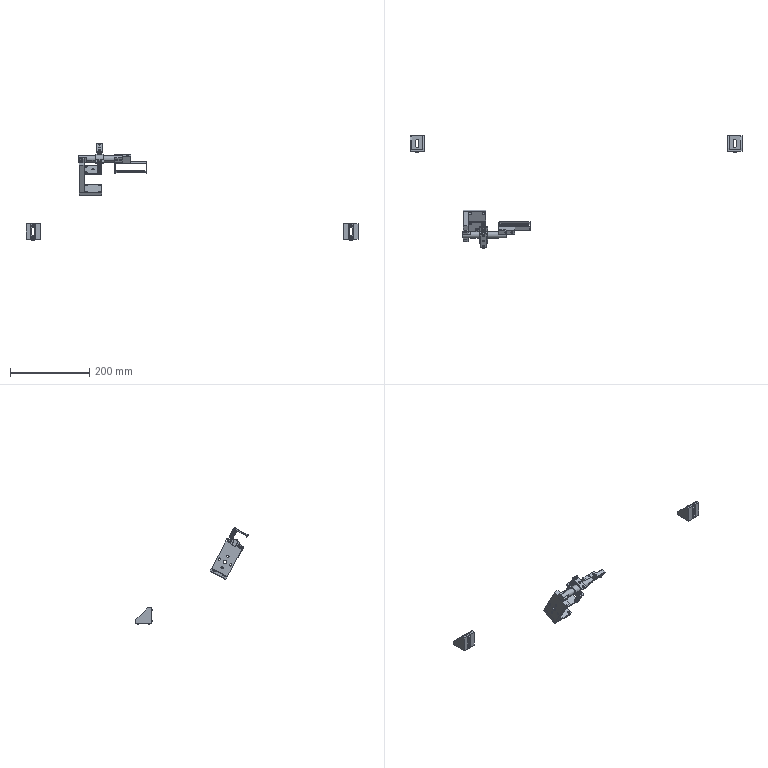Assembly | SolidWorks | mm | 21 component files | 21 solids | 520 faces | box 836 x 284.58 x 242.95 mm | volume 129529 mm3 | plane 300 | cylinder 172 | cone 24 | torus 18 | spline 6 | commonest cylinder face diameters 6 x22 10 x14 5 x12 4 x12 5.5 x12 6.5 x12 3 x10 7 x10
Bill of materials:
ABB11-G408-4040AngleBracket | 2 |  | Right-angle corner-block bracket with a triangular, chamfered side profile. Each of its two perpendicular faces has an obround slot, and small rectangular locating tabs stick out from those faces.
BladeConnectingRod | 1 |  | Solid cylindrical shaft or rod with a flat milled on each end. One flat has a single larger cross hole; the other has two smaller holes.
clevis pins with head gb | 1 |  | Headed cylindrical pin with a domed, rounded head, a plain shank, and one transverse cross hole near the chamfered tip, consistent with a clevis-style pin.
hexagon socket head cap screws gb | 4 |  | Socket-head cap-screw-shaped part: a cylindrical head with a hexagonal socket and a plain cylindrical shank.
RotaryCylinderFixingPlate | 1 |  | Thick rectangular plate or block with two narrow tabs extending from one edge, each with a hole through its thickness. The main face has a pattern of one larger centre hole and four smaller surrounding holes.
SDACylinderFixingPlate | 1 |  | Flat rectangular plate with sharp corners and six through-holes in two rows of three. The holes near one edge are smaller than the others.
SDACylinderPushPlate | 1 |  | Thin flat rectangular plate with rounded corners, four corner through-holes and one larger central through-hole.
SDACylinderSpringPressurePlate | 1 |  | Flat elongated strip/link plate with rounded corners: two larger through-holes near the ends and one smaller through-hole at the centre.
split pins | 1 |  | Split pin (cotter-pin-like) shape: a wire folded back on itself, with a looped eye at one end and two legs of unequal length with flat inner faces.
Spring | 2 |  | Helical coil spring with round wire, constant diameter and open, evenly spaced coils.
Spring | 1 |  | Open-coiled cylindrical helix shaped like a coil spring: a single continuous wire wound at a constant coil diameter and roughly even pitch, about 11-12 turns, with plain cut ends.
SpringSnap | 2 |  | Formed sheet-metal saddle/pipe-clamp shape: a central semicircular arch with flat flanges on both sides, each flange having an obround slot.
Blade | 1 |  | Long, narrow bent sheet strip with a V-shaped end profile and a rounded bend. A long rectangular opening runs along most of its length, and small narrow tabs extend at each end.
CutterFixingBlock | 1 |  | Solid rectangular block with sharp edges. It has two round holes in one long face and two round holes in an adjacent perpendicular face. One hole from each pair breaks into a hole from the other pair.
ToolHolder | 1 |  | Strap of thin bent sheet with a U or channel shape. A long flat middle section has two round holes and is bent at both ends into legs on the same side. Each leg narrows to a rounded tip with one small round hole.
Mates:
1. coincident | RotaryCylinderFixingPlate-1 face at (-267.317, -3.29, 87.691) dir (0, 0.4648, -0.8854) | SDACylinderFixingPlate-1 face at (-251.317, 16.632, 98.15) dir (0, -0.4648, 0.8854)
2. coincident | RotaryCylinderFixingPlate-1 face at (-267.317, -5.28, 188.295) dir (0, 0.8854, 0.4648) | SDACylinderFixingPlate-1 face at (-223.317, 40.272, 101.525) dir (0, 0.8854, 0.4648)
3. coincident | RotaryCylinderFixingPlate-1 face at (-279.317, -4.285, 137.993) dir (-1, 0, 0) | SDACylinderFixingPlate-1 face at (-279.317, 0.429, 80.608) dir (-1, 0, 0)
4. coincident | RotaryCylinderFixingPlate-1 face at (-279.317, -36.136, 187.908) dir (0, 0.8854, 0.4648) | BladeConnectingRod-1 face at (-260.317, -23.937, 164.67) dir (0, -0.8854, -0.4648)
5. concentric | RotaryCylinderFixingPlate-1 face at (-273.317, -13.559, 177.172) dir (0, 0.8854, 0.4648) r 3 | BladeConnectingRod-1 face at (-273.317, -26.84, 170.2) dir (0, -0.8854, -0.4648) r 3
6. concentric | ToolHolderAssembly-1/CutterFixingBlock-1 face at (-185.317, -17.986, 174.848) dir (0, -0.8854, -0.4648) r 2.5 | BladeConnectingRod-1 face at (-185.317, -26.84, 170.2) dir (0, -0.8854, -0.4648) r 1.65
7. concentric | ToolHolderAssembly-1/CutterFixingBlock-1 face at (-175.317, -17.986, 174.848) dir (0, -0.8854, -0.4648) r 2.5 | BladeConnectingRod-1 face at (-175.317, -26.84, 170.2) dir (0, -0.8854, -0.4648) r 1.65
8. parallel | RotaryCylinderFixingPlate-1 face at (-267.317, -5.28, 188.295) dir (0, 0.8854, 0.4648) | SDACylinderPushPlate-1 face at (-223.317, 9.286, 155.17) dir (0, 0.8854, 0.4648)
9. concentric | SDACylinderPushPlate-1 face at (-228.317, -20.308, 136.245) dir (0, 0.4648, -0.8854) r 2.5 | SDACylinderSpringPressurePlate-1 face at (-228.317, -50.986, 194.681) dir (0, -0.4648, 0.8854) r 3.25
10. distance | SDACylinderPushPlate-1 face at (-245.317, -8.422, 145.873) dir (0, -0.4648, 0.8854) | SDACylinderSpringPressurePlate-1 face at (-228.317, -36.311, 198.998) dir (0, 0.4648, -0.8854)
11. concentric | hexagon socket head cap screws gb-2 face at (-228.317, -21.635, 203.314) dir (0, -0.4648, 0.8854) r 0.8 | SDACylinderSpringPressurePlate-1 face at (-228.317, -24.424, 208.626) dir (0, -0.4648, 0.8854) r 3.25
12. coincident | SDACylinderSpringPressurePlate-1 face at (-228.317, -37.705, 201.654) dir (0, -0.4648, 0.8854) | hexagon socket head cap screws gb-2 face at (-228.317, -24.424, 208.626) dir (0, 0.4648, -0.8854)
13. concentric | SDACylinderPushPlate-1 face at (-228.317, 6.254, 150.189) dir (0, 0.4648, -0.8854) r 2.5 | hexagon socket head cap screws gb-2 face at (-228.317, -21.635, 203.314) dir (0, -0.4648, 0.8854) r 0.8
14. slot | SpringSnap-1 face at (-225.822, -2.314, 174.04) dir (0, -0.8854, -0.4648) | hexagon socket head cap screws gb-2 face at (-228.317, -21.635, 203.314) dir (0, -0.4648, 0.8854) r 0.8
15. slot | SpringSnap-1 face at (-226.423, -35.074, 156.842) dir (0, 0.8854, 0.4648) | hexagon socket head cap screws gb-3 face at (-228.317, -51.739, 187.51) dir (0, -0.4648, 0.8854) r 0.8
16. coincident | SpringSnap-1 face at (-218.322, -29.496, 168.805) dir (0, 0.4648, -0.8854) | SpringSnap-2 face at (-238.322, -15.329, 176.242) dir (0, -0.4648, 0.8854)
17. coincident | SpringSnap-1 face at (-218.322, -42.777, 161.833) dir (0, -0.8854, -0.4648) | SpringSnap-2 face at (-238.322, -42.777, 161.833) dir (0, -0.8854, -0.4648)
18. coincident | SpringSnap-1 face at (-218.322, -32.159, 170.286) dir (1, 0, 0) | SpringSnap-2 face at (-218.322, -30.333, 165.275) dir (1, 0, 0)
19. coincident | ToolHolderAssembly-1/CutterFixingBlock-1 face at (-150.317, -20.45, 179.542) dir (0, -0.8854, -0.4648) | BladeConnectingRod-1 face at (-190.317, -15.083, 169.319) dir (0, 0.8854, 0.4648)
20. concentric | BladeConnectingRod-1 face at (-273.317, -26.84, 170.2) dir (0, -0.8854, -0.4648) r 3 | clevis pins with head gb-1 face at (-273.317, 5.327, 187.087) dir (0, 0.8854, 0.4648) r 1.5
21. coincident | RotaryCylinderFixingPlate-1 face at (-279.317, -16.348, 182.485) dir (0, 0.8854, 0.4648) | clevis pins with head gb-1 face at (-274.637, -13.889, 177.802) dir (0, -0.8854, -0.4648)
22. concentric | clevis pins with head gb-1 face at (-271.115, -20.091, 172.404) dir (-0.8805, -0.2203, 0.4197) r 0.87 | split pins-2 face at (-262.72, -17.99, 168.403) dir (-0.8805, -0.2203, 0.4197) r 0.25
23. concentric | hexagon socket head cap screws gb-2 face at (-228.317, -21.635, 203.314) dir (0, -0.4648, 0.8854) r 0.8 | Spring-1 sketch segment at (-228.317, 4.976, 152.623) dir (0, -0.4648, 0.8854) r 4.5
24. coincident | SDACylinderPushPlate-1 face at (-245.317, -8.422, 145.873) dir (0, -0.4648, 0.8854) | Spring-1 face at (-237.317, -0.1812, 150.199) dir (0, 0.4648, -0.8854)
25. concentric | hexagon socket head cap screws gb-3 face at (-228.317, -51.739, 187.51) dir (0, -0.4648, 0.8854) r 0.8 | Spring-2 sketch segment at (-228.317, -25.128, 136.819) dir (0, -0.4648, 0.8854) r 4.5
26. coincident | SDACylinderPushPlate-1 face at (-245.317, -8.422, 145.873) dir (0, -0.4648, 0.8854) | Spring-2 face at (-237.317, -30.285, 134.395) dir (0, 0.4648, -0.8854)
27. concentric | hexagon socket head cap screws gb-2 face at (-228.317, -21.635, 203.314) dir (0, -0.4648, 0.8854) r 0.8 | Spring-3 sketch segment at (-228.317, -23.146, 206.192) dir (0, 0.4648, -0.8854) r 4.5
28. coincident | SDACylinderSpringPressurePlate-1 face at (-228.317, -36.311, 198.998) dir (0, 0.4648, -0.8854) | Spring-3 face at (-238.89, -23.98, 205.471) dir (0, -0.4648, 0.8854)
29. concentric | BladeConnectingRod-1 face at (-170.317, -22.413, 172.524) dir (-1, 0, 0) r 8 | SpringSnap-1 face at (-218.322, -22.413, 172.524) dir (-1, 0, 0) r 8
30. tangent | RotaryCylinderFixingPlate-1 face at (-279.317, -23.121, 163.117) dir (0, -0.4648, 0.8854) | BladeConnectingRod-1 face at (-170.317, -22.413, 172.524) dir (-1, 0, 0) r 8
31. concentric | Blade-1 face at (-29.739, 17.848, 39.396) dir (0, 0, -1) r 1.25 | ToolHolder-1 face at (-29.739, 17.848, -41.604) dir (0, 0, 1) r 1.25
32. coincident | Blade-1 face at (-30.989, 16.598, 37.396) dir (0, 0, 1) | ToolHolder-1 face at (-25.471, 44.002, 37.396) dir (0, 0, -1)
33. coincident | CutterFixingBlock-1 face at (-17.155, 63.923, -41.604) dir (0, 0, -1) | ToolHolder-1 face at (-25.471, 44.002, -41.604) dir (0, 0, -1)
34. coincident | CutterFixingBlock-1 face at (-25.31, 44.989, -21.604) dir (-0.161, -0.9869, 0) | ToolHolder-1 face at (-25.31, 44.989, -1.604) dir (0.161, 0.9869, 0)
35. coincident | CutterFixingBlock-1 face at (-27.025, 65.533, -1.604) dir (-0.9869, 0.161, 0) | ToolHolder-1 face at (-30.245, 45.794, 38.396) dir (-0.9869, 0.161, 0)
36. concentric | CutterFixingBlock-1 face at (-25.31, 44.989, -23.604) dir (-0.161, -0.9869, 0) r 2 | hexagon socket head cap screws gb-1 face at (-24.505, 49.924, -23.604) dir (-0.161, -0.9869, 0) r 0.8
37. coincident | ToolHolder-1 face at (-25.471, 44.002, -1.604) dir (-0.161, -0.9869, 0) | hexagon socket head cap screws gb-1 face at (-25.471, 44.002, -23.604) dir (0.161, 0.9869, 0)
38. concentric | CutterFixingBlock-1 face at (-25.31, 44.989, -8.604) dir (-0.161, -0.9869, 0) r 2 | hexagon socket head cap screws gb-2 face at (-24.505, 49.924, -8.604) dir (-0.161, -0.9869, 0) r 0.8
39. coincident | ToolHolder-1 face at (-25.471, 44.002, -1.604) dir (-0.161, -0.9869, 0) | hexagon socket head cap screws gb-2 face at (-25.471, 44.002, -8.604) dir (0.161, 0.9869, 0)